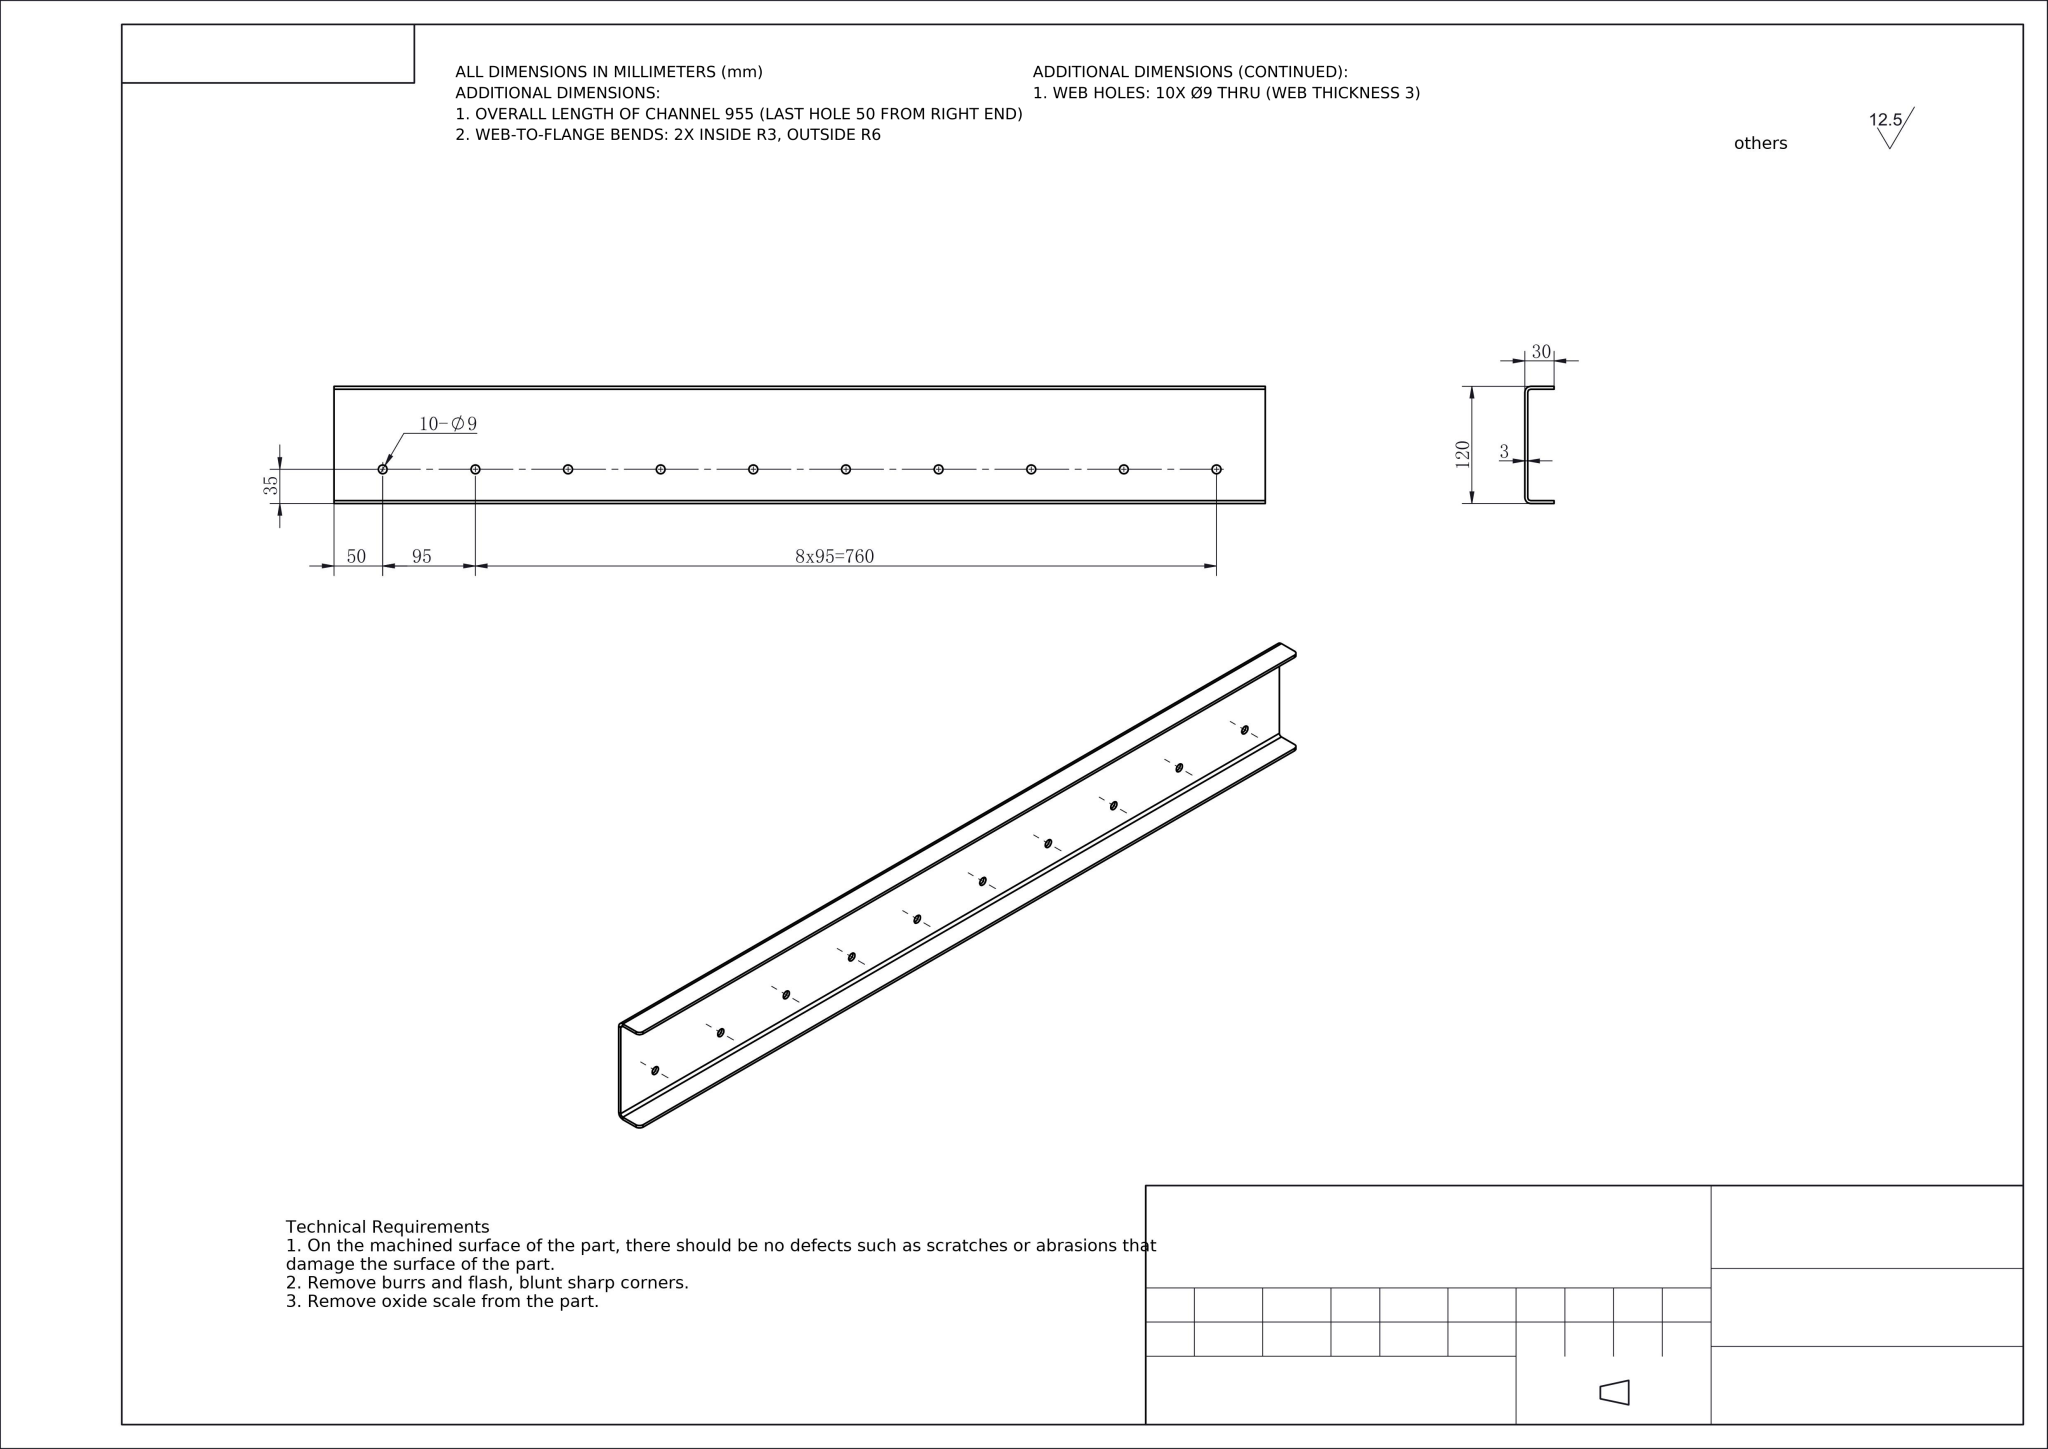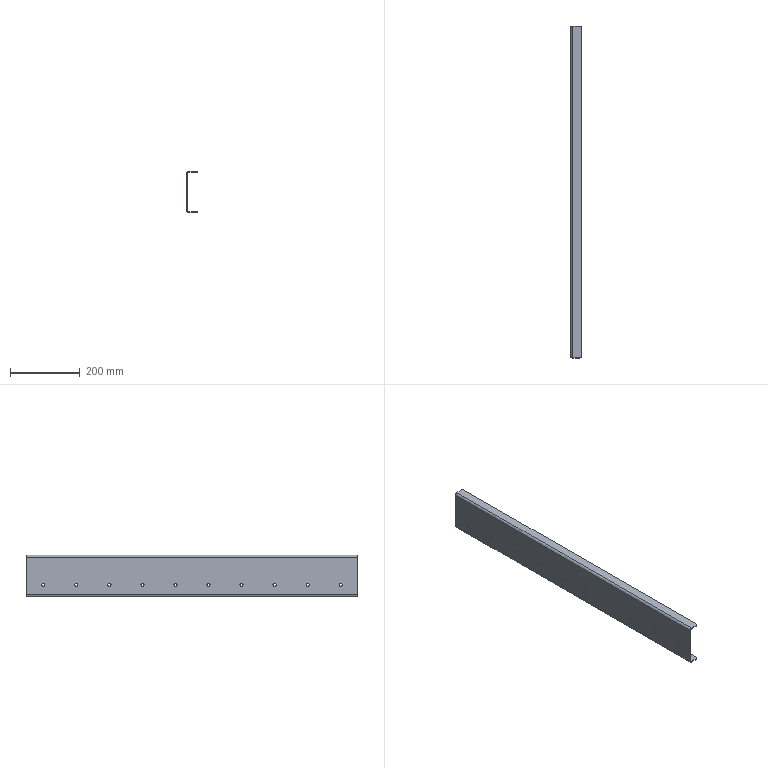Part | NX | mm | 1 solid | 46 faces | box 30 x 955 x 120 mm | volume 485470 mm3 | cylinder 28 | plane 18 | commonest cylinder face diameters 9 x20 10 x4 6 x2 12 x2